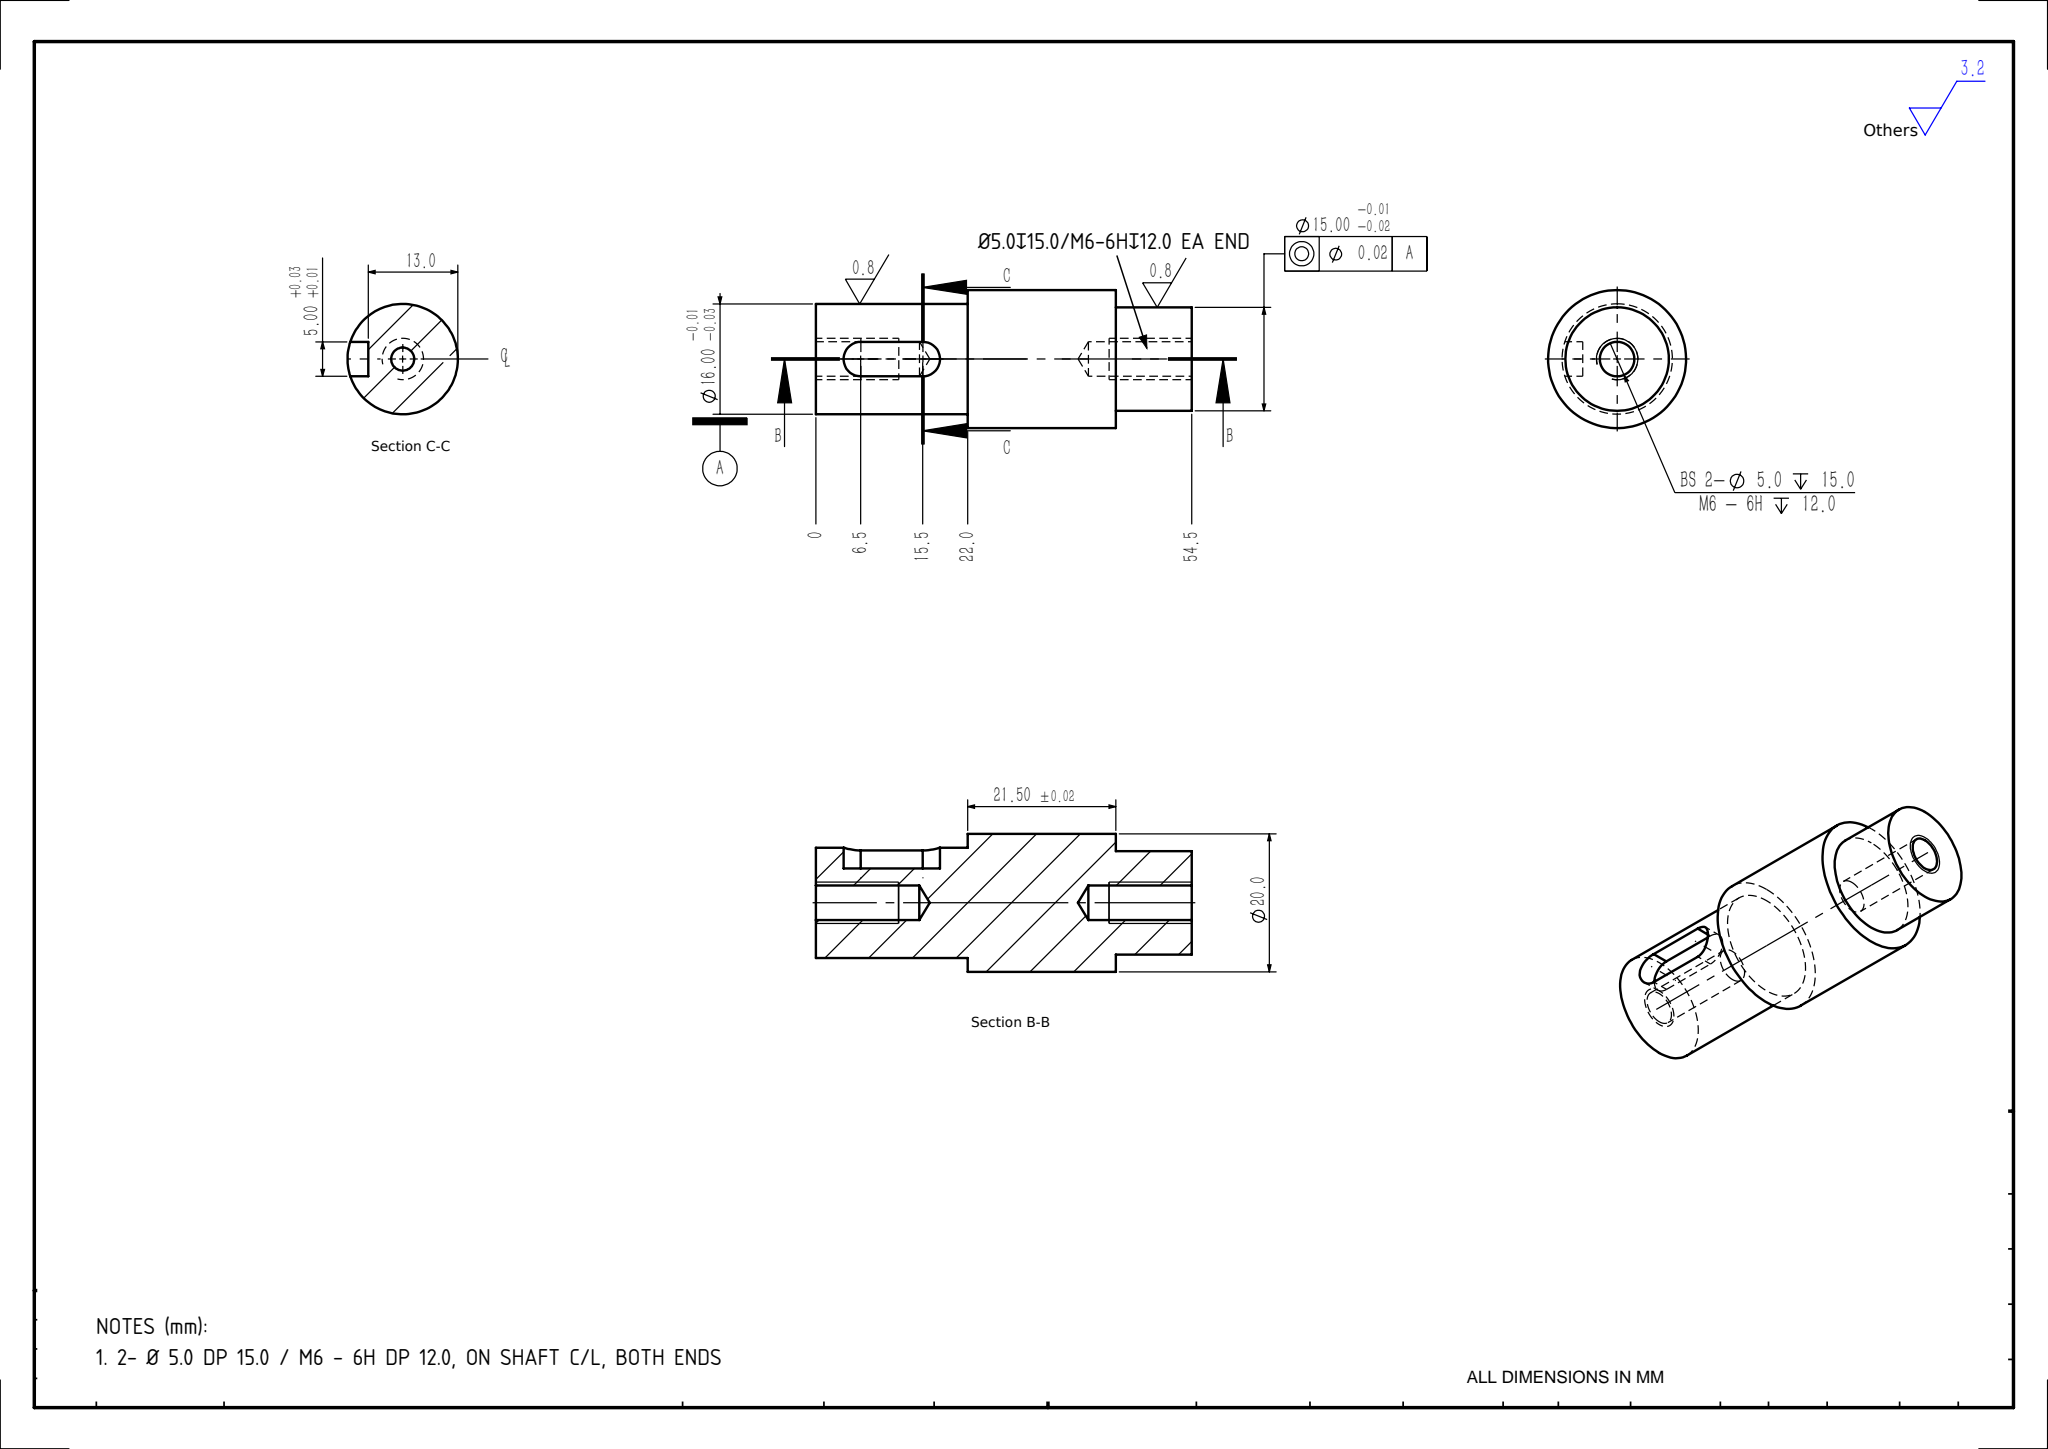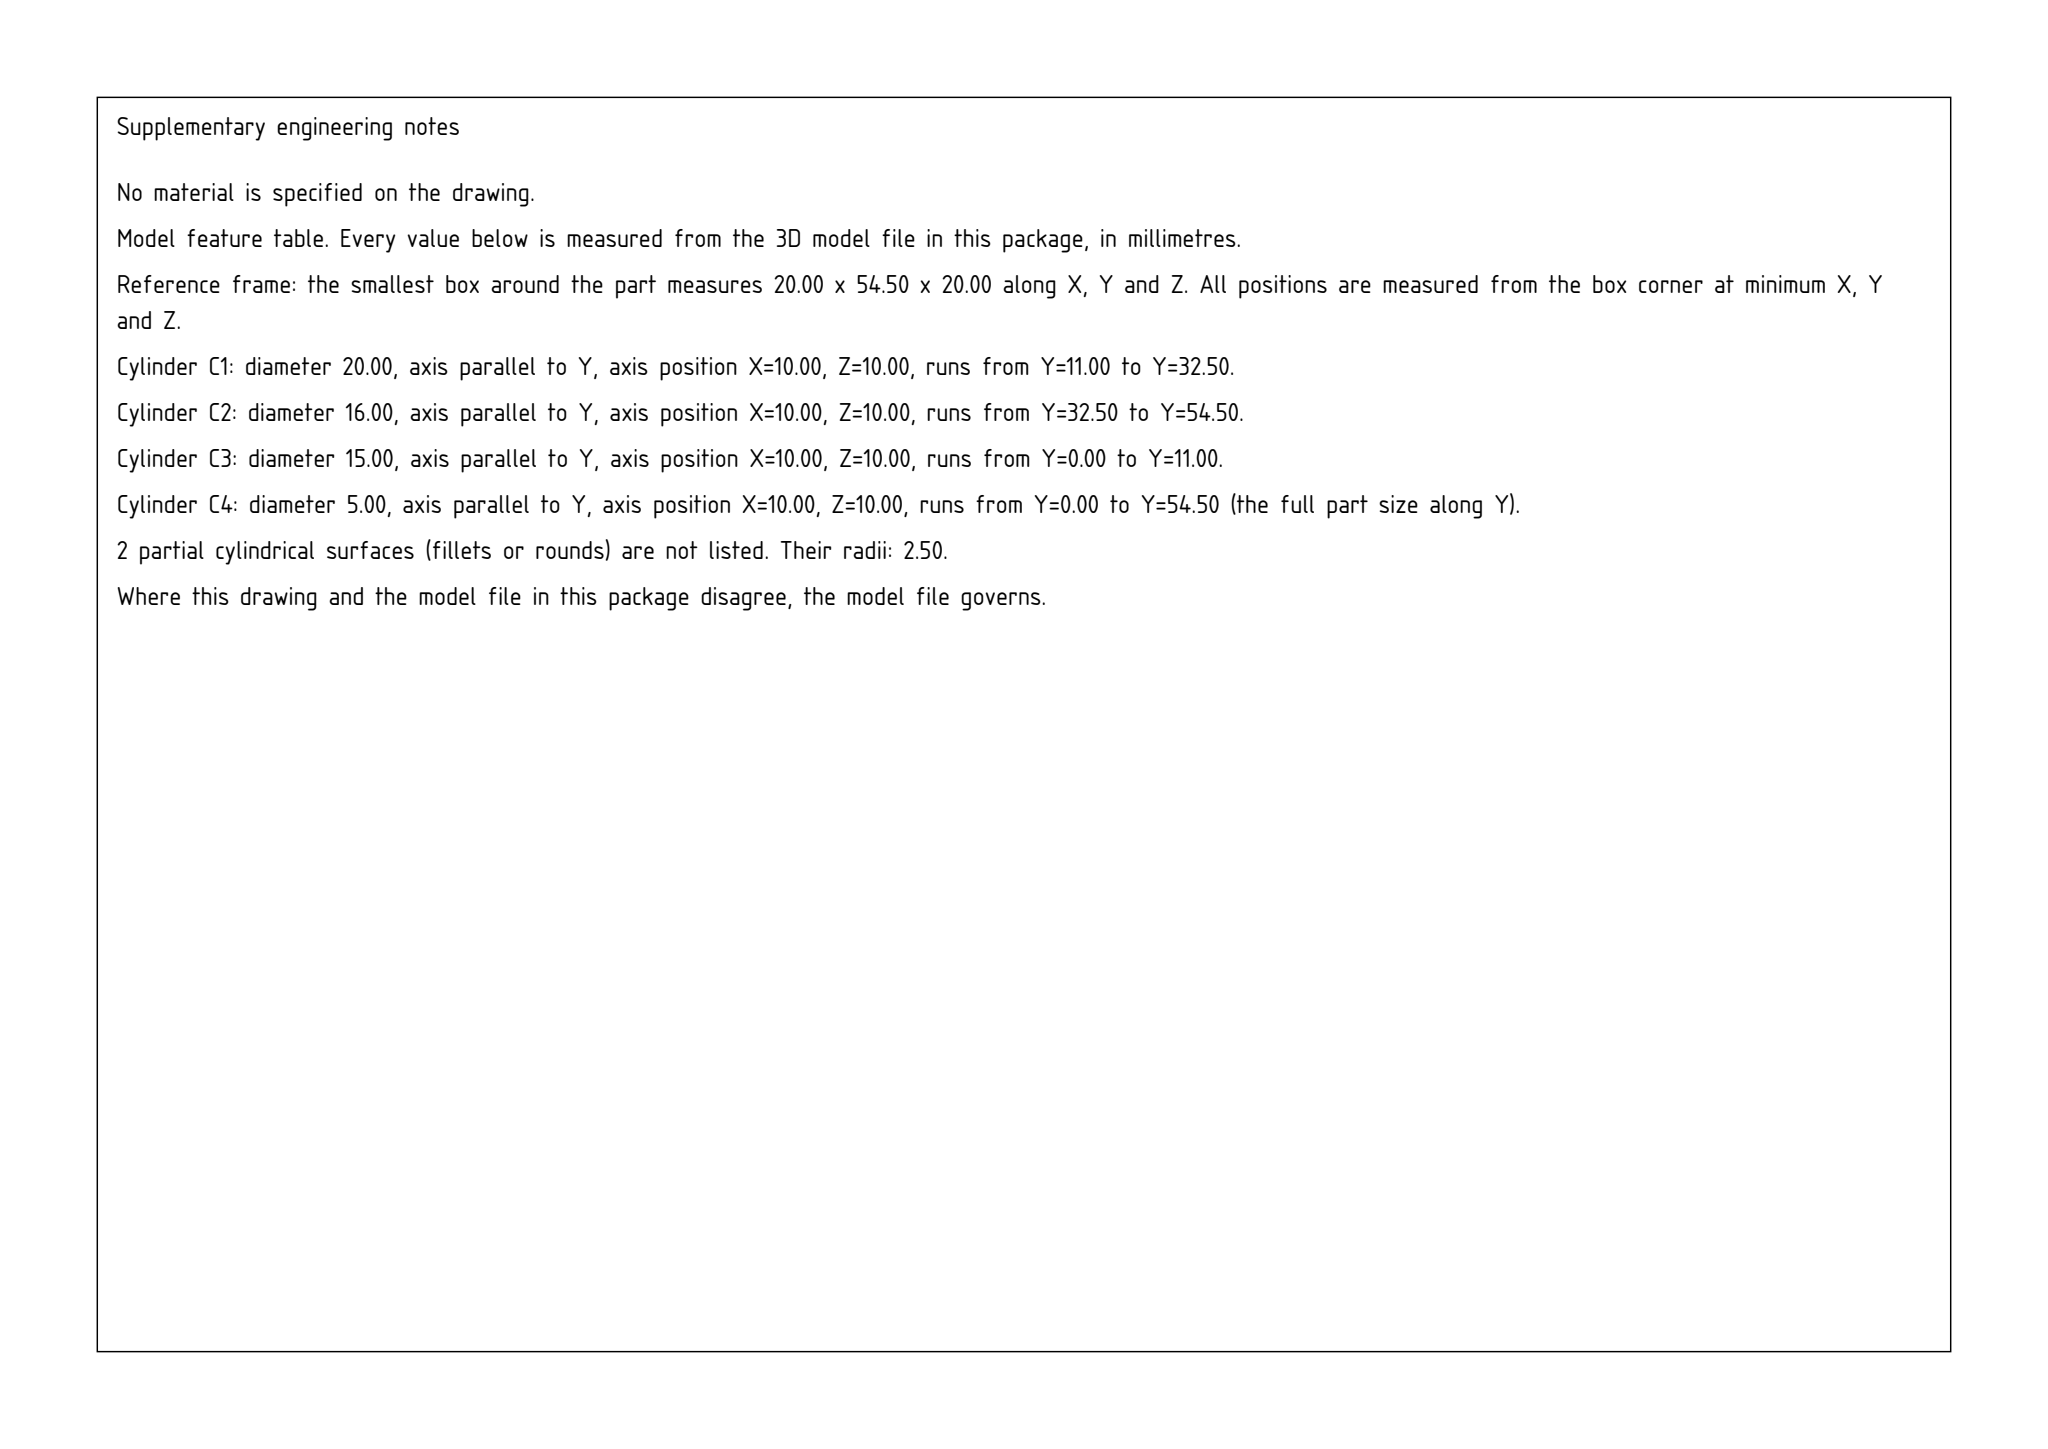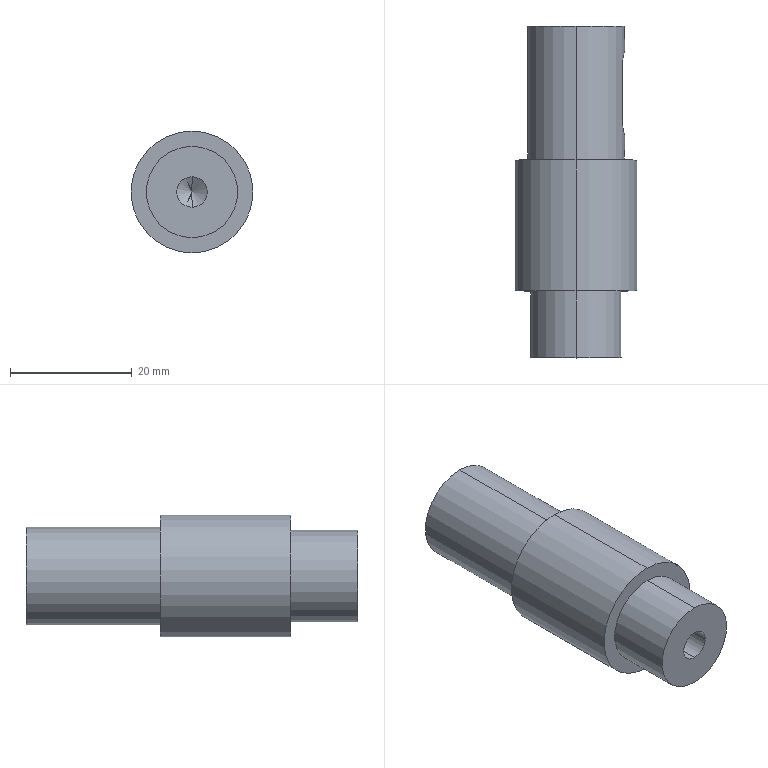Part | SolidWorks | mm | 1 solid | 23 faces | box 20 x 54.5 x 20 mm | volume 12327 mm3 | cylinder 12 | plane 7 | cone 4 | commonest cylinder face diameters 5 x6 15 x2 16 x2 20 x2
Drawing notes:
2- Ø 5.0 DP 15.0 / M6 - 6H DP 12.0, ON SHAFT C/L, BOTH ENDS | from the solid: Two Ø5.0 bores on Y axis at [10,10]: y 0->15 and y 39.5->54.5 (15 deep each), with 118° drill points; threaded M6 depth 12 per callout
2- Ø5.0 DP 15.0 / M6-6H DP 12.0, ONE EA END (DELETE "BS") | from the solid: Two Ø5.0 y-axis bores: y 0.0-15.0 and y 39.5-54.5 (15 deep each), both on axis x=10,z=10; 118° drill points at Ø5.0
build123d program:
from build123d import *

# Parameters (mm, degrees)
SKETCH1_R             = 8
BOSS_EXTRUDE1_DEPTH   = 22
SKETCH2_R             = 10
BOSS_EXTRUDE2_DEPTH   = 32.5
CUT_EXTRUDE1_START    = -11
SKETCH3_R             = 10
SKETCH3_R_2           = 7.5
CUT_EXTRUDE1_DEPTH    = 11
M6_TAPPED_HOLE1_D     = 5
M6_TAPPED_HOLE1_DEPTH = 15
M6_TAPPED_HOLE1_TIP   = 1.502
M6_TAPPED_HOLE2_D     = 5
M6_TAPPED_HOLE2_DEPTH = 15
M6_TAPPED_HOLE2_TIP   = 1.502
CUT_EXTRUDE2_DEPTH    = 3


with BuildPart() as part:
    # Sketch1 → Boss-Extrude1 (new body)
    with BuildSketch(Plane(origin=(0, 0, 0), x_dir=(1, 0, 0), z_dir=(0, 1, 0))):
        with Locations(Location((0, 0, 0), (0, 0, 270))):
            Circle(SKETCH1_R)
    extrude(amount=BOSS_EXTRUDE1_DEPTH)

    # Sketch2 → Boss-Extrude2 (add)
    with BuildSketch(Plane.XZ):
        with Locations(Location((0, 0, 0), (0, 0, 270))):
            Circle(SKETCH2_R)
    extrude(amount=BOSS_EXTRUDE2_DEPTH)

    # Sketch3 → Cut-Extrude1 (cut)
    with BuildSketch(Plane.XZ.offset(32.5).offset(CUT_EXTRUDE1_START)):
        with Locations(Location((0, 0, 0), (0, 0, 270))):
            Circle(SKETCH3_R)
        with Locations(Location((0, 0, 0), (0, 0, 270))):
            Circle(SKETCH3_R_2, mode=Mode.SUBTRACT)
    extrude(amount=CUT_EXTRUDE1_DEPTH, mode=Mode.SUBTRACT)

    # M6 Tapped Hole1
    with Locations(Plane(origin=(0, 22, 0), x_dir=(1, 0, 0), z_dir=(0, 1, 0))):
        with Locations((0, 0)):
            Hole(M6_TAPPED_HOLE1_D / 2, depth=M6_TAPPED_HOLE1_DEPTH)
            with Locations((0, 0, -(M6_TAPPED_HOLE1_DEPTH + M6_TAPPED_HOLE1_TIP / 2))):  # 118° drill point
                Cone(0, M6_TAPPED_HOLE1_D / 2, M6_TAPPED_HOLE1_TIP, mode=Mode.SUBTRACT)

    # M6 Tapped Hole2
    with Locations(Plane(origin=(0, -32.5, 0), x_dir=(-1, 0, 0), z_dir=(0, -1, 0))):
        with Locations((0, 0)):
            Hole(M6_TAPPED_HOLE2_D / 2, depth=M6_TAPPED_HOLE2_DEPTH)
            with Locations((0, 0, -(M6_TAPPED_HOLE2_DEPTH + M6_TAPPED_HOLE2_TIP / 2))):  # 118° drill point
                Cone(0, M6_TAPPED_HOLE2_D / 2, M6_TAPPED_HOLE2_TIP, mode=Mode.SUBTRACT)

    # Sketch11 → Cut-Extrude2 (cut)
    with BuildSketch(Plane(origin=(8, 0, 0), x_dir=(0, 0, -1), z_dir=(1, 0, 0))):
        with BuildLine():
            Line((-2.5, 6.5), (-2.5, 15.5))
            ThreePointArc((-2.5, 15.5), (0, 18), (2.5, 15.5))
            Line((2.5, 15.5), (2.5, 6.5))
            ThreePointArc((2.5, 6.5), (0, 4), (-2.5, 6.5))
        make_face()
    extrude(amount=-CUT_EXTRUDE2_DEPTH, mode=Mode.SUBTRACT)


solid = part.part
STEP:
#1=CARTESIAN_POINT('',(0.,-17.5,2.5));
#2=VERTEX_POINT('',#1);
#3=CARTESIAN_POINT('',(0.,-17.5,-2.5));
#4=VERTEX_POINT('',#3);
#5=CARTESIAN_POINT('',(0.,-17.5,0.));
#6=DIRECTION('',(0.,-1.,0.));
#7=DIRECTION('',(0.,0.,-1.));
#8=AXIS2_PLACEMENT_3D('',#5,#6,#7);
#9=CIRCLE('',#8,2.5);
#10=EDGE_CURVE('',#2,#4,#9,.T.);
#11=ORIENTED_EDGE('',*,*,#10,.F.);
#12=CARTESIAN_POINT('',(0.,-32.5,2.5));
#13=VERTEX_POINT('',#12);
#14=CARTESIAN_POINT('',(0.,-32.5,2.5));
#15=DIRECTION('',(0.,-1.,0.));
#16=VECTOR('',#15,1000.);
#17=LINE('',#14,#16);
#18=EDGE_CURVE('',#2,#13,#17,.T.);
#19=ORIENTED_EDGE('',*,*,#18,.T.);
#20=CARTESIAN_POINT('',(0.,-32.5,-2.5));
#21=VERTEX_POINT('',#20);
#22=CARTESIAN_POINT('',(0.,-32.5,0.));
#23=DIRECTION('',(0.,-1.,0.));
#24=DIRECTION('',(0.,0.,-1.));
#25=AXIS2_PLACEMENT_3D('',#22,#23,#24);
#26=CIRCLE('',#25,2.5);
#27=EDGE_CURVE('',#13,#21,#26,.T.);
#28=ORIENTED_EDGE('',*,*,#27,.T.);
#29=CARTESIAN_POINT('',(0.,-32.5,-2.5));
#30=DIRECTION('',(0.,-1.,0.));
#31=VECTOR('',#30,1000.);
#32=LINE('',#29,#31);
#33=EDGE_CURVE('',#4,#21,#32,.T.);
#34=ORIENTED_EDGE('',*,*,#33,.F.);
#35=EDGE_LOOP('',(#11,#19,#28,#34));
#36=FACE_OUTER_BOUND('',#35,.T.);
#37=CARTESIAN_POINT('',(0.,-32.5,0.));
#38=DIRECTION('',(0.,-1.,0.));
#39=DIRECTION('',(0.,0.,-1.));
#40=AXIS2_PLACEMENT_3D('',#37,#38,#39);
#41=CYLINDRICAL_SURFACE('',#40,2.5);
#42=ADVANCED_FACE('',(#36),#41,.F.);
#43=CARTESIAN_POINT('',(-0.,-15.998,0.));
#44=VERTEX_POINT('',#43);
#45=CARTESIAN_POINT('',(0.,-17.5,-2.5));
#46=DIRECTION('',(0.,-0.515,-0.8572));
#47=VECTOR('',#46,1000.);
#48=LINE('',#45,#47);
#49=EDGE_CURVE('',#44,#4,#48,.T.);
#50=ORIENTED_EDGE('',*,*,#49,.F.);
#51=CARTESIAN_POINT('',(0.,-17.5,2.5));
#52=DIRECTION('',(0.,-0.515,0.8572));
#53=VECTOR('',#52,1000.);
#54=LINE('',#51,#53);
#55=EDGE_CURVE('',#44,#2,#54,.T.);
#56=ORIENTED_EDGE('',*,*,#55,.T.);
#57=ORIENTED_EDGE('',*,*,#10,.T.);
#58=EDGE_LOOP('',(#50,#56,#57));
#59=FACE_OUTER_BOUND('',#58,.T.);
#60=CARTESIAN_POINT('',(0.,-17.5,0.));
#61=DIRECTION('',(0.,-1.,0.));
#62=DIRECTION('',(0.,0.,-1.));
#63=AXIS2_PLACEMENT_3D('',#60,#61,#62);
#64=CONICAL_SURFACE('',#63,2.5,1.03);
#65=ADVANCED_FACE('',(#59),#64,.F.);
#66=CARTESIAN_POINT('',(0.,7.,-2.5));
#67=VERTEX_POINT('',#66);
#68=CARTESIAN_POINT('',(0.,7.,2.5));
#69=VERTEX_POINT('',#68);
#70=CARTESIAN_POINT('',(0.,7.,0.));
#71=DIRECTION('',(0.,1.,0.));
#72=DIRECTION('',(0.,0.,1.));
#73=AXIS2_PLACEMENT_3D('',#70,#71,#72);
#74=CIRCLE('',#73,2.5);
#75=EDGE_CURVE('',#67,#69,#74,.T.);
#76=ORIENTED_EDGE('',*,*,#75,.F.);
#77=CARTESIAN_POINT('',(0.,22.,-2.5));
#78=VERTEX_POINT('',#77);
#79=CARTESIAN_POINT('',(0.,22.,-2.5));
#80=DIRECTION('',(0.,1.,0.));
#81=VECTOR('',#80,1000.);
#82=LINE('',#79,#81);
#83=EDGE_CURVE('',#67,#78,#82,.T.);
#84=ORIENTED_EDGE('',*,*,#83,.T.);
#85=CARTESIAN_POINT('',(0.,22.,2.5));
#86=VERTEX_POINT('',#85);
#87=CARTESIAN_POINT('',(0.,22.,0.));
#88=DIRECTION('',(0.,1.,0.));
#89=DIRECTION('',(0.,0.,1.));
#90=AXIS2_PLACEMENT_3D('',#87,#88,#89);
#91=CIRCLE('',#90,2.5);
#92=EDGE_CURVE('',#78,#86,#91,.T.);
#93=ORIENTED_EDGE('',*,*,#92,.T.);
#94=CARTESIAN_POINT('',(0.,22.,2.5));
#95=DIRECTION('',(0.,1.,0.));
#96=VECTOR('',#95,1000.);
#97=LINE('',#94,#96);
#98=EDGE_CURVE('',#69,#86,#97,.T.);
#99=ORIENTED_EDGE('',*,*,#98,.F.);
#100=EDGE_LOOP('',(#76,#84,#93,#99));
#101=FACE_OUTER_BOUND('',#100,.T.);
#102=CARTESIAN_POINT('',(0.,22.,0.));
#103=DIRECTION('',(0.,1.,0.));
#104=DIRECTION('',(0.,0.,1.));
#105=AXIS2_PLACEMENT_3D('',#102,#103,#104);
#106=CYLINDRICAL_SURFACE('',#105,2.5);
#107=ADVANCED_FACE('',(#101),#106,.F.);
#108=CARTESIAN_POINT('',(-0.,5.498,0.));
#109=VERTEX_POINT('',#108);
#110=CARTESIAN_POINT('',(0.,7.,2.5));
#111=DIRECTION('',(0.,0.515,0.8572));
#112=VECTOR('',#111,1000.);
#113=LINE('',#110,#112);
#114=EDGE_CURVE('',#109,#69,#113,.T.);
#115=ORIENTED_EDGE('',*,*,#114,.F.);
#116=CARTESIAN_POINT('',(0.,7.,-2.5));
#117=DIRECTION('',(0.,0.515,-0.8572));
#118=VECTOR('',#117,1000.);
#119=LINE('',#116,#118);
#120=EDGE_CURVE('',#109,#67,#119,.T.);
#121=ORIENTED_EDGE('',*,*,#120,.T.);
#122=ORIENTED_EDGE('',*,*,#75,.T.);
#123=EDGE_LOOP('',(#115,#121,#122));
#124=FACE_OUTER_BOUND('',#123,.T.);
#125=CARTESIAN_POINT('',(0.,7.,0.));
#126=DIRECTION('',(0.,1.,0.));
#127=DIRECTION('',(0.,0.,1.));
#128=AXIS2_PLACEMENT_3D('',#125,#126,#127);
#129=CONICAL_SURFACE('',#128,2.5,1.03);
#130=ADVANCED_FACE('',(#124),#129,.F.);
#131=CARTESIAN_POINT('',(0.,-21.5,-7.5));
#132=VERTEX_POINT('',#131);
#133=CARTESIAN_POINT('',(0.,-21.5,7.5));
#134=VERTEX_POINT('',#133);
#135=CARTESIAN_POINT('',(0.,-21.5,0.));
#136=DIRECTION('',(0.,-1.,0.));
#137=DIRECTION('',(0.,0.,-1.));
#138=AXIS2_PLACEMENT_3D('',#135,#136,#137);
#139=CIRCLE('',#138,7.5);
#140=EDGE_CURVE('',#132,#134,#139,.T.);
#141=ORIENTED_EDGE('',*,*,#140,.T.);
#142=CARTESIAN_POINT('',(0.,-32.5,7.5));
#143=VERTEX_POINT('',#142);
#144=CARTESIAN_POINT('',(0.,-21.5,7.5));
#145=DIRECTION('',(0.,-1.,0.));
#146=VECTOR('',#145,1000.);
#147=LINE('',#144,#146);
#148=EDGE_CURVE('',#134,#143,#147,.T.);
#149=ORIENTED_EDGE('',*,*,#148,.T.);
#150=CARTESIAN_POINT('',(0.,-32.5,-7.5));
#151=VERTEX_POINT('',#150);
#152=CARTESIAN_POINT('',(0.,-32.5,0.));
#153=DIRECTION('',(0.,-1.,0.));
#154=DIRECTION('',(0.,0.,-1.));
#155=AXIS2_PLACEMENT_3D('',#152,#153,#154);
#156=CIRCLE('',#155,7.5);
#157=EDGE_CURVE('',#151,#143,#156,.T.);
#158=ORIENTED_EDGE('',*,*,#157,.F.);
#159=CARTESIAN_POINT('',(0.,-21.5,-7.5));
#160=DIRECTION('',(0.,-1.,0.));
#161=VECTOR('',#160,1000.);
#162=LINE('',#159,#161);
#163=EDGE_CURVE('',#132,#151,#162,.T.);
#164=ORIENTED_EDGE('',*,*,#163,.F.);
#165=EDGE_LOOP('',(#141,#149,#158,#164));
#166=FACE_OUTER_BOUND('',#165,.T.);
#167=CARTESIAN_POINT('',(0.,-21.5,0.));
#168=DIRECTION('',(0.,-1.,0.));
#169=DIRECTION('',(0.,0.,-1.));
#170=AXIS2_PLACEMENT_3D('',#167,#168,#169);
#171=CYLINDRICAL_SURFACE('',#170,7.5);
#172=ADVANCED_FACE('',(#166),#171,.T.);
#173=CARTESIAN_POINT('',(7.599,6.5,2.5));
#174=VERTEX_POINT('',#173);
#175=CARTESIAN_POINT('',(7.599,15.5,2.5));
#176=VERTEX_POINT('',#175);
#177=CARTESIAN_POINT('',(7.599,22.,2.5));
#178=DIRECTION('',(0.,1.,0.));
#179=VECTOR('',#178,1000.);
#180=LINE('',#177,#179);
#181=EDGE_CURVE('',#174,#176,#180,.T.);
#182=ORIENTED_EDGE('',*,*,#181,.T.);
#183=CARTESIAN_POINT('',(7.599,15.5,-2.5));
#184=VERTEX_POINT('',#183);
#185=CARTESIAN_POINT('',(7.599,15.5,2.5));
#186=CARTESIAN_POINT('',(7.599,15.666,2.5));
#187=CARTESIAN_POINT('',(7.605,15.83,2.484));
#188=CARTESIAN_POINT('',(7.625,16.15,2.419));
#189=CARTESIAN_POINT('',(7.641,16.31,2.371));
#190=CARTESIAN_POINT('',(7.679,16.612,2.245));
#191=CARTESIAN_POINT('',(7.701,16.755,2.168));
#192=CARTESIAN_POINT('',(7.75,17.026,1.987));
#193=CARTESIAN_POINT('',(7.776,17.153,1.882));
#194=CARTESIAN_POINT('',(7.854,17.497,1.539));
#195=CARTESIAN_POINT('',(7.906,17.683,1.262));
#196=CARTESIAN_POINT('',(7.96,17.87,0.8114));
#197=CARTESIAN_POINT('',(7.975,17.919,0.6527));
#198=CARTESIAN_POINT('',(7.995,17.984,0.3296));
#199=CARTESIAN_POINT('',(8.,18.,0.1667));
#200=CARTESIAN_POINT('',(8.,18.,-0.1617));
#201=CARTESIAN_POINT('',(7.995,17.984,-0.3285));
#202=CARTESIAN_POINT('',(7.975,17.92,-0.6499));
#203=CARTESIAN_POINT('',(7.961,17.872,-0.8063));
#204=CARTESIAN_POINT('',(7.924,17.746,-1.11));
#205=CARTESIAN_POINT('',(7.902,17.668,-1.255));
#206=CARTESIAN_POINT('',(7.855,17.488,-1.525));
#207=CARTESIAN_POINT('',(7.828,17.383,-1.652));
#208=CARTESIAN_POINT('',(7.776,17.153,-1.883));
#209=CARTESIAN_POINT('',(7.75,17.028,-1.985));
#210=CARTESIAN_POINT('',(7.702,16.758,-2.166));
#211=CARTESIAN_POINT('',(7.679,16.612,-2.245));
#212=CARTESIAN_POINT('',(7.641,16.311,-2.37));
#213=CARTESIAN_POINT('',(7.626,16.155,-2.418));
#214=CARTESIAN_POINT('',(7.605,15.832,-2.483));
#215=CARTESIAN_POINT('',(7.599,15.666,-2.5));
#216=CARTESIAN_POINT('',(7.599,15.5,-2.5));
#217=B_SPLINE_CURVE_WITH_KNOTS('',3,(#185,#186,#187,#188,#189,#190,#191,#192,#193,#194,#195,#196,#197,#198,#199,#200,#201,#202,#203,#204,#205,#206,#207,#208,#209,#210,#211,#212,#213,#214,#215,#216),.UNSPECIFIED.,.F.,.F.,(4,2,2,2,2,2,2,2,2,2,2,2,2,2,2,4),(0.,0.0004914,0.0009828,0.001474,0.001966,0.002949,0.00344,0.003931,0.004423,0.004914,0.005406,0.005897,0.006388,0.00688,0.007371,0.007863),.UNSPECIFIED.);
#218=EDGE_CURVE('',#176,#184,#217,.T.);
#219=ORIENTED_EDGE('',*,*,#218,.T.);
#220=CARTESIAN_POINT('',(7.599,6.5,-2.5));
#221=VERTEX_POINT('',#220);
#222=CARTESIAN_POINT('',(7.599,22.,-2.5));
#223=DIRECTION('',(0.,-1.,0.));
#224=VECTOR('',#223,1000.);
#225=LINE('',#222,#224);
#226=EDGE_CURVE('',#184,#221,#225,.T.);
#227=ORIENTED_EDGE('',*,*,#226,.T.);
#228=CARTESIAN_POINT('',(7.599,6.5,-2.5));
#229=CARTESIAN_POINT('',(7.599,6.334,-2.5));
#230=CARTESIAN_POINT('',(7.605,6.17,-2.484));
#231=CARTESIAN_POINT('',(7.625,5.85,-2.419));
#232=CARTESIAN_POINT('',(7.641,5.69,-2.371));
#233=CARTESIAN_POINT('',(7.679,5.388,-2.245));
#234=CARTESIAN_POINT('',(7.701,5.245,-2.168));
#235=CARTESIAN_POINT('',(7.75,4.974,-1.987));
#236=CARTESIAN_POINT('',(7.776,4.847,-1.882));
#237=CARTESIAN_POINT('',(7.854,4.503,-1.539));
#238=CARTESIAN_POINT('',(7.906,4.317,-1.262));
#239=CARTESIAN_POINT('',(7.96,4.13,-0.8114));
#240=CARTESIAN_POINT('',(7.975,4.081,-0.6527));
#241=CARTESIAN_POINT('',(7.995,4.016,-0.3296));
#242=CARTESIAN_POINT('',(8.,4.,-0.1667));
#243=CARTESIAN_POINT('',(8.,4.,0.1617));
#244=CARTESIAN_POINT('',(7.995,4.016,0.3285));
#245=CARTESIAN_POINT('',(7.975,4.08,0.6499));
#246=CARTESIAN_POINT('',(7.961,4.128,0.8063));
#247=CARTESIAN_POINT('',(7.924,4.254,1.11));
#248=CARTESIAN_POINT('',(7.902,4.332,1.255));
#249=CARTESIAN_POINT('',(7.855,4.512,1.525));
#250=CARTESIAN_POINT('',(7.828,4.617,1.652));
#251=CARTESIAN_POINT('',(7.776,4.847,1.883));
#252=CARTESIAN_POINT('',(7.75,4.972,1.985));
#253=CARTESIAN_POINT('',(7.702,5.242,2.166));
#254=CARTESIAN_POINT('',(7.679,5.388,2.245));
#255=CARTESIAN_POINT('',(7.641,5.689,2.37));
#256=CARTESIAN_POINT('',(7.626,5.845,2.418));
#257=CARTESIAN_POINT('',(7.605,6.168,2.483));
#258=CARTESIAN_POINT('',(7.599,6.334,2.5));
#259=CARTESIAN_POINT('',(7.599,6.5,2.5));
#260=B_SPLINE_CURVE_WITH_KNOTS('',3,(#228,#229,#230,#231,#232,#233,#234,#235,#236,#237,#238,#239,#240,#241,#242,#243,#244,#245,#246,#247,#248,#249,#250,#251,#252,#253,#254,#255,#256,#257,#258,#259),.UNSPECIFIED.,.F.,.F.,(4,2,2,2,2,2,2,2,2,2,2,2,2,2,2,4),(0.,0.0004914,0.0009828,0.001474,0.001966,0.002949,0.00344,0.003931,0.004423,0.004914,0.005406,0.005897,0.006388,0.00688,0.007371,0.007863),.UNSPECIFIED.);
#261=EDGE_CURVE('',#221,#174,#260,.T.);
#262=ORIENTED_EDGE('',*,*,#261,.T.);
#263=EDGE_LOOP('',(#182,#219,#227,#262));
#264=FACE_BOUND('',#263,.T.);
#265=CARTESIAN_POINT('',(0.,22.,8.));
#266=VERTEX_POINT('',#265);
#267=CARTESIAN_POINT('',(0.,22.,-8.));
#268=VERTEX_POINT('',#267);
#269=CARTESIAN_POINT('',(0.,22.,0.));
#270=DIRECTION('',(0.,1.,0.));
#271=DIRECTION('',(0.,0.,1.));
#272=AXIS2_PLACEMENT_3D('',#269,#270,#271);
#273=CIRCLE('',#272,8.);
#274=EDGE_CURVE('',#266,#268,#273,.T.);
#275=ORIENTED_EDGE('',*,*,#274,.F.);
#276=CARTESIAN_POINT('',(0.,0.,8.));
#277=VERTEX_POINT('',#276);
#278=CARTESIAN_POINT('',(0.,22.,8.));
#279=DIRECTION('',(0.,-1.,0.));
#280=VECTOR('',#279,1000.);
#281=LINE('',#278,#280);
#282=EDGE_CURVE('',#266,#277,#281,.T.);
#283=ORIENTED_EDGE('',*,*,#282,.T.);
#284=CARTESIAN_POINT('',(0.,0.,-8.));
#285=VERTEX_POINT('',#284);
#286=CARTESIAN_POINT('',(0.,0.,0.));
#287=DIRECTION('',(0.,-1.,0.));
#288=DIRECTION('',(0.,0.,-1.));
#289=AXIS2_PLACEMENT_3D('',#286,#287,#288);
#290=CIRCLE('',#289,8.);
#291=EDGE_CURVE('',#285,#277,#290,.T.);
#292=ORIENTED_EDGE('',*,*,#291,.F.);
#293=CARTESIAN_POINT('',(0.,22.,-8.));
#294=DIRECTION('',(0.,-1.,0.));
#295=VECTOR('',#294,1000.);
#296=LINE('',#293,#295);
#297=EDGE_CURVE('',#268,#285,#296,.T.);
#298=ORIENTED_EDGE('',*,*,#297,.F.);
#299=EDGE_LOOP('',(#275,#283,#292,#298));
#300=FACE_OUTER_BOUND('',#299,.T.);
#301=CARTESIAN_POINT('',(0.,22.,0.));
#302=DIRECTION('',(0.,-1.,0.));
#303=DIRECTION('',(0.,0.,-1.));
#304=AXIS2_PLACEMENT_3D('',#301,#302,#303);
#305=CYLINDRICAL_SURFACE('',#304,8.);
#306=ADVANCED_FACE('',(#264,#300),#305,.T.);
#307=CARTESIAN_POINT('',(0.,-21.5,-10.));
#308=VERTEX_POINT('',#307);
#309=CARTESIAN_POINT('',(0.,-21.5,10.));
#310=VERTEX_POINT('',#309);
#311=CARTESIAN_POINT('',(0.,-21.5,0.));
#312=DIRECTION('',(0.,-1.,0.));
#313=DIRECTION('',(0.,0.,-1.));
#314=AXIS2_PLACEMENT_3D('',#311,#312,#313);
#315=CIRCLE('',#314,10.);
#316=EDGE_CURVE('',#308,#310,#315,.T.);
#317=ORIENTED_EDGE('',*,*,#316,.F.);
#318=CARTESIAN_POINT('',(0.,0.,-10.));
#319=VERTEX_POINT('',#318);
#320=CARTESIAN_POINT('',(0.,-32.5,-10.));
#321=DIRECTION('',(0.,1.,0.));
#322=VECTOR('',#321,1000.);
#323=LINE('',#320,#322);
#324=EDGE_CURVE('',#308,#319,#323,.T.);
#325=ORIENTED_EDGE('',*,*,#324,.T.);
#326=CARTESIAN_POINT('',(0.,0.,10.));
#327=VERTEX_POINT('',#326);
#328=CARTESIAN_POINT('',(0.,0.,0.));
#329=DIRECTION('',(0.,-1.,0.));
#330=DIRECTION('',(0.,0.,-1.));
#331=AXIS2_PLACEMENT_3D('',#328,#329,#330);
#332=CIRCLE('',#331,10.);
#333=EDGE_CURVE('',#319,#327,#332,.T.);
#334=ORIENTED_EDGE('',*,*,#333,.T.);
#335=CARTESIAN_POINT('',(0.,-32.5,10.));
#336=DIRECTION('',(0.,1.,0.));
#337=VECTOR('',#336,1000.);
#338=LINE('',#335,#337);
#339=EDGE_CURVE('',#310,#327,#338,.T.);
#340=ORIENTED_EDGE('',*,*,#339,.F.);
#341=EDGE_LOOP('',(#317,#325,#334,#340));
#342=FACE_OUTER_BOUND('',#341,.T.);
#343=CARTESIAN_POINT('',(0.,-32.5,0.));
#344=DIRECTION('',(0.,1.,0.));
#345=DIRECTION('',(0.,0.,1.));
#346=AXIS2_PLACEMENT_3D('',#343,#344,#345);
#347=CYLINDRICAL_SURFACE('',#346,10.);
#348=ADVANCED_FACE('',(#342),#347,.T.);
#349=ORIENTED_EDGE('',*,*,#324,.F.);
#350=CARTESIAN_POINT('',(0.,-21.5,0.));
#351=DIRECTION('',(0.,-1.,0.));
#352=DIRECTION('',(0.,0.,-1.));
#353=AXIS2_PLACEMENT_3D('',#350,#351,#352);
#354=CIRCLE('',#353,10.);
#355=EDGE_CURVE('',#310,#308,#354,.T.);
#356=ORIENTED_EDGE('',*,*,#355,.F.);
#357=ORIENTED_EDGE('',*,*,#339,.T.);
#358=CARTESIAN_POINT('',(0.,0.,0.));
#359=DIRECTION('',(0.,-1.,0.));
#360=DIRECTION('',(0.,0.,-1.));
#361=AXIS2_PLACEMENT_3D('',#358,#359,#360);
#362=CIRCLE('',#361,10.);
#363=EDGE_CURVE('',#327,#319,#362,.T.);
#364=ORIENTED_EDGE('',*,*,#363,.T.);
#365=EDGE_LOOP('',(#349,#356,#357,#364));
#366=FACE_OUTER_BOUND('',#365,.T.);
#367=CARTESIAN_POINT('',(0.,-32.5,0.));
#368=DIRECTION('',(0.,1.,0.));
#369=DIRECTION('',(0.,0.,1.));
#370=AXIS2_PLACEMENT_3D('',#367,#368,#369);
#371=CYLINDRICAL_SURFACE('',#370,10.);
#372=ADVANCED_FACE('',(#366),#371,.T.);
#373=ORIENTED_EDGE('',*,*,#282,.F.);
#374=CARTESIAN_POINT('',(0.,22.,0.));
#375=DIRECTION('',(0.,1.,0.));
#376=DIRECTION('',(0.,0.,1.));
#377=AXIS2_PLACEMENT_3D('',#374,#375,#376);
#378=CIRCLE('',#377,8.);
#379=EDGE_CURVE('',#268,#266,#378,.T.);
#380=ORIENTED_EDGE('',*,*,#379,.F.);
#381=ORIENTED_EDGE('',*,*,#297,.T.);
#382=CARTESIAN_POINT('',(0.,0.,0.));
#383=DIRECTION('',(0.,-1.,0.));
#384=DIRECTION('',(0.,0.,-1.));
#385=AXIS2_PLACEMENT_3D('',#382,#383,#384);
#386=CIRCLE('',#385,8.);
#387=EDGE_CURVE('',#277,#285,#386,.T.);
#388=ORIENTED_EDGE('',*,*,#387,.F.);
#389=EDGE_LOOP('',(#373,#380,#381,#388));
#390=FACE_OUTER_BOUND('',#389,.T.);
#391=CARTESIAN_POINT('',(0.,22.,0.));
#392=DIRECTION('',(0.,-1.,0.));
#393=DIRECTION('',(0.,0.,-1.));
#394=AXIS2_PLACEMENT_3D('',#391,#392,#393);
#395=CYLINDRICAL_SURFACE('',#394,8.);
#396=ADVANCED_FACE('',(#390),#395,.T.);
#397=CARTESIAN_POINT('',(0.,22.,0.));
#398=DIRECTION('',(0.,1.,0.));
#399=DIRECTION('',(0.,0.,1.));
#400=AXIS2_PLACEMENT_3D('',#397,#398,#399);
#401=CIRCLE('',#400,2.5);
#402=EDGE_CURVE('',#86,#78,#401,.T.);
#403=ORIENTED_EDGE('',*,*,#402,.F.);
#404=ORIENTED_EDGE('',*,*,#92,.F.);
#405=EDGE_LOOP('',(#403,#404));
#406=FACE_BOUND('',#405,.T.);
#407=ORIENTED_EDGE('',*,*,#379,.T.);
#408=ORIENTED_EDGE('',*,*,#274,.T.);
#409=EDGE_LOOP('',(#407,#408));
#410=FACE_OUTER_BOUND('',#409,.T.);
#411=CARTESIAN_POINT('',(0.,22.,0.));
#412=DIRECTION('',(0.,1.,0.));
#413=DIRECTION('',(0.,0.,1.));
#414=AXIS2_PLACEMENT_3D('',#411,#412,#413);
#415=PLANE('',#414);
#416=ADVANCED_FACE('',(#406,#410),#415,.T.);
#417=ORIENTED_EDGE('',*,*,#291,.T.);
#418=ORIENTED_EDGE('',*,*,#387,.T.);
#419=EDGE_LOOP('',(#417,#418));
#420=FACE_BOUND('',#419,.T.);
#421=ORIENTED_EDGE('',*,*,#363,.F.);
#422=ORIENTED_EDGE('',*,*,#333,.F.);
#423=EDGE_LOOP('',(#421,#422));
#424=FACE_OUTER_BOUND('',#423,.T.);
#425=CARTESIAN_POINT('',(0.,0.,0.));
#426=DIRECTION('',(0.,-1.,0.));
#427=DIRECTION('',(0.,0.,-1.));
#428=AXIS2_PLACEMENT_3D('',#425,#426,#427);
#429=PLANE('',#428);
#430=ADVANCED_FACE('',(#420,#424),#429,.F.);
#431=ORIENTED_EDGE('',*,*,#140,.F.);
#432=CARTESIAN_POINT('',(0.,-21.5,0.));
#433=DIRECTION('',(0.,-1.,0.));
#434=DIRECTION('',(0.,0.,-1.));
#435=AXIS2_PLACEMENT_3D('',#432,#433,#434);
#436=CIRCLE('',#435,7.5);
#437=EDGE_CURVE('',#134,#132,#436,.T.);
#438=ORIENTED_EDGE('',*,*,#437,.F.);
#439=EDGE_LOOP('',(#431,#438));
#440=FACE_BOUND('',#439,.T.);
#441=ORIENTED_EDGE('',*,*,#355,.T.);
#442=ORIENTED_EDGE('',*,*,#316,.T.);
#443=EDGE_LOOP('',(#441,#442));
#444=FACE_OUTER_BOUND('',#443,.T.);
#445=CARTESIAN_POINT('',(0.,-21.5,0.));
#446=DIRECTION('',(0.,-1.,0.));
#447=DIRECTION('',(0.,0.,-1.));
#448=AXIS2_PLACEMENT_3D('',#445,#446,#447);
#449=PLANE('',#448);
#450=ADVANCED_FACE('',(#440,#444),#449,.T.);
#451=ORIENTED_EDGE('',*,*,#148,.F.);
#452=ORIENTED_EDGE('',*,*,#437,.T.);
#453=ORIENTED_EDGE('',*,*,#163,.T.);
#454=CARTESIAN_POINT('',(0.,-32.5,0.));
#455=DIRECTION('',(0.,-1.,0.));
#456=DIRECTION('',(0.,0.,-1.));
#457=AXIS2_PLACEMENT_3D('',#454,#455,#456);
#458=CIRCLE('',#457,7.5);
#459=EDGE_CURVE('',#143,#151,#458,.T.);
#460=ORIENTED_EDGE('',*,*,#459,.F.);
#461=EDGE_LOOP('',(#451,#452,#453,#460));
#462=FACE_OUTER_BOUND('',#461,.T.);
#463=CARTESIAN_POINT('',(0.,-21.5,0.));
#464=DIRECTION('',(0.,-1.,0.));
#465=DIRECTION('',(0.,0.,-1.));
#466=AXIS2_PLACEMENT_3D('',#463,#464,#465);
#467=CYLINDRICAL_SURFACE('',#466,7.5);
#468=ADVANCED_FACE('',(#462),#467,.T.);
#469=CARTESIAN_POINT('',(0.,-32.5,0.));
#470=DIRECTION('',(0.,-1.,0.));
#471=DIRECTION('',(0.,0.,-1.));
#472=AXIS2_PLACEMENT_3D('',#469,#470,#471);
#473=CIRCLE('',#472,2.5);
#474=EDGE_CURVE('',#21,#13,#473,.T.);
#475=ORIENTED_EDGE('',*,*,#474,.F.);
#476=ORIENTED_EDGE('',*,*,#27,.F.);
#477=EDGE_LOOP('',(#475,#476));
#478=FACE_BOUND('',#477,.T.);
#479=ORIENTED_EDGE('',*,*,#157,.T.);
#480=ORIENTED_EDGE('',*,*,#459,.T.);
#481=EDGE_LOOP('',(#479,#480));
#482=FACE_OUTER_BOUND('',#481,.T.);
#483=CARTESIAN_POINT('',(0.,-32.5,0.));
#484=DIRECTION('',(0.,-1.,0.));
#485=DIRECTION('',(0.,0.,-1.));
#486=AXIS2_PLACEMENT_3D('',#483,#484,#485);
#487=PLANE('',#486);
#488=ADVANCED_FACE('',(#478,#482),#487,.T.);
#489=ORIENTED_EDGE('',*,*,#120,.F.);
#490=ORIENTED_EDGE('',*,*,#114,.T.);
#491=CARTESIAN_POINT('',(0.,7.,0.));
#492=DIRECTION('',(0.,1.,0.));
#493=DIRECTION('',(0.,0.,1.));
#494=AXIS2_PLACEMENT_3D('',#491,#492,#493);
#495=CIRCLE('',#494,2.5);
#496=EDGE_CURVE('',#69,#67,#495,.T.);
#497=ORIENTED_EDGE('',*,*,#496,.T.);
#498=EDGE_LOOP('',(#489,#490,#497));
#499=FACE_OUTER_BOUND('',#498,.T.);
#500=CARTESIAN_POINT('',(0.,7.,0.));
#501=DIRECTION('',(0.,1.,0.));
#502=DIRECTION('',(0.,0.,1.));
#503=AXIS2_PLACEMENT_3D('',#500,#501,#502);
#504=CONICAL_SURFACE('',#503,2.5,1.03);
#505=ADVANCED_FACE('',(#499),#504,.F.);
#506=ORIENTED_EDGE('',*,*,#83,.F.);
#507=ORIENTED_EDGE('',*,*,#496,.F.);
#508=ORIENTED_EDGE('',*,*,#98,.T.);
#509=ORIENTED_EDGE('',*,*,#402,.T.);
#510=EDGE_LOOP('',(#506,#507,#508,#509));
#511=FACE_OUTER_BOUND('',#510,.T.);
#512=CARTESIAN_POINT('',(0.,22.,0.));
#513=DIRECTION('',(0.,1.,0.));
#514=DIRECTION('',(0.,0.,1.));
#515=AXIS2_PLACEMENT_3D('',#512,#513,#514);
#516=CYLINDRICAL_SURFACE('',#515,2.5);
#517=ADVANCED_FACE('',(#511),#516,.F.);
#518=ORIENTED_EDGE('',*,*,#55,.F.);
#519=ORIENTED_EDGE('',*,*,#49,.T.);
#520=CARTESIAN_POINT('',(0.,-17.5,0.));
#521=DIRECTION('',(0.,-1.,0.));
#522=DIRECTION('',(0.,0.,-1.));
#523=AXIS2_PLACEMENT_3D('',#520,#521,#522);
#524=CIRCLE('',#523,2.5);
#525=EDGE_CURVE('',#4,#2,#524,.T.);
#526=ORIENTED_EDGE('',*,*,#525,.T.);
#527=EDGE_LOOP('',(#518,#519,#526));
#528=FACE_OUTER_BOUND('',#527,.T.);
#529=CARTESIAN_POINT('',(0.,-17.5,0.));
#530=DIRECTION('',(0.,-1.,0.));
#531=DIRECTION('',(0.,0.,-1.));
#532=AXIS2_PLACEMENT_3D('',#529,#530,#531);
#533=CONICAL_SURFACE('',#532,2.5,1.03);
#534=ADVANCED_FACE('',(#528),#533,.F.);
#535=ORIENTED_EDGE('',*,*,#18,.F.);
#536=ORIENTED_EDGE('',*,*,#525,.F.);
#537=ORIENTED_EDGE('',*,*,#33,.T.);
#538=ORIENTED_EDGE('',*,*,#474,.T.);
#539=EDGE_LOOP('',(#535,#536,#537,#538));
#540=FACE_OUTER_BOUND('',#539,.T.);
#541=CARTESIAN_POINT('',(0.,-32.5,0.));
#542=DIRECTION('',(0.,-1.,0.));
#543=DIRECTION('',(0.,0.,-1.));
#544=AXIS2_PLACEMENT_3D('',#541,#542,#543);
#545=CYLINDRICAL_SURFACE('',#544,2.5);
#546=ADVANCED_FACE('',(#540),#545,.F.);
#547=CARTESIAN_POINT('',(5.,6.5,-2.5));
#548=VERTEX_POINT('',#547);
#549=CARTESIAN_POINT('',(5.,6.5,-2.5));
#550=DIRECTION('',(1.,0.,0.));
#551=VECTOR('',#550,1000.);
#552=LINE('',#549,#551);
#553=EDGE_CURVE('',#548,#221,#552,.T.);
#554=ORIENTED_EDGE('',*,*,#553,.F.);
#555=CARTESIAN_POINT('',(5.,6.5,2.5));
#556=VERTEX_POINT('',#555);
#557=CARTESIAN_POINT('',(5.,6.5,0.));
#558=DIRECTION('',(1.,0.,0.));
#559=DIRECTION('',(0.,0.,-1.));
#560=AXIS2_PLACEMENT_3D('',#557,#558,#559);
#561=CIRCLE('',#560,2.5);
#562=EDGE_CURVE('',#556,#548,#561,.T.);
#563=ORIENTED_EDGE('',*,*,#562,.F.);
#564=CARTESIAN_POINT('',(5.,6.5,2.5));
#565=DIRECTION('',(1.,0.,0.));
#566=VECTOR('',#565,1000.);
#567=LINE('',#564,#566);
#568=EDGE_CURVE('',#556,#174,#567,.T.);
#569=ORIENTED_EDGE('',*,*,#568,.T.);
#570=ORIENTED_EDGE('',*,*,#261,.F.);
#571=EDGE_LOOP('',(#554,#563,#569,#570));
#572=FACE_OUTER_BOUND('',#571,.T.);
#573=CARTESIAN_POINT('',(5.,6.5,0.));
#574=DIRECTION('',(1.,0.,0.));
#575=DIRECTION('',(0.,0.,-1.));
#576=AXIS2_PLACEMENT_3D('',#573,#574,#575);
#577=CYLINDRICAL_SURFACE('',#576,2.5);
#578=ADVANCED_FACE('',(#572),#577,.F.);
#579=ORIENTED_EDGE('',*,*,#568,.F.);
#580=CARTESIAN_POINT('',(5.,15.5,2.5));
#581=VERTEX_POINT('',#580);
#582=CARTESIAN_POINT('',(5.,6.5,2.5));
#583=DIRECTION('',(0.,-1.,0.));
#584=VECTOR('',#583,1000.);
#585=LINE('',#582,#584);
#586=EDGE_CURVE('',#581,#556,#585,.T.);
#587=ORIENTED_EDGE('',*,*,#586,.F.);
#588=CARTESIAN_POINT('',(5.,15.5,2.5));
#589=DIRECTION('',(1.,0.,0.));
#590=VECTOR('',#589,1000.);
#591=LINE('',#588,#590);
#592=EDGE_CURVE('',#581,#176,#591,.T.);
#593=ORIENTED_EDGE('',*,*,#592,.T.);
#594=ORIENTED_EDGE('',*,*,#181,.F.);
#595=EDGE_LOOP('',(#579,#587,#593,#594));
#596=FACE_OUTER_BOUND('',#595,.T.);
#597=CARTESIAN_POINT('',(5.,6.5,2.5));
#598=DIRECTION('',(0.,0.,1.));
#599=DIRECTION('',(1.,0.,0.));
#600=AXIS2_PLACEMENT_3D('',#597,#598,#599);
#601=PLANE('',#600);
#602=ADVANCED_FACE('',(#596),#601,.F.);
#603=ORIENTED_EDGE('',*,*,#592,.F.);
#604=CARTESIAN_POINT('',(5.,15.5,-2.5));
#605=VERTEX_POINT('',#604);
#606=CARTESIAN_POINT('',(5.,15.5,0.));
#607=DIRECTION('',(1.,0.,0.));
#608=DIRECTION('',(0.,0.,-1.));
#609=AXIS2_PLACEMENT_3D('',#606,#607,#608);
#610=CIRCLE('',#609,2.5);
#611=EDGE_CURVE('',#605,#581,#610,.T.);
#612=ORIENTED_EDGE('',*,*,#611,.F.);
#613=CARTESIAN_POINT('',(5.,15.5,-2.5));
#614=DIRECTION('',(1.,0.,0.));
#615=VECTOR('',#614,1000.);
#616=LINE('',#613,#615);
#617=EDGE_CURVE('',#605,#184,#616,.T.);
#618=ORIENTED_EDGE('',*,*,#617,.T.);
#619=ORIENTED_EDGE('',*,*,#218,.F.);
#620=EDGE_LOOP('',(#603,#612,#618,#619));
#621=FACE_OUTER_BOUND('',#620,.T.);
#622=CARTESIAN_POINT('',(5.,15.5,0.));
#623=DIRECTION('',(1.,0.,0.));
#624=DIRECTION('',(0.,0.,-1.));
#625=AXIS2_PLACEMENT_3D('',#622,#623,#624);
#626=CYLINDRICAL_SURFACE('',#625,2.5);
#627=ADVANCED_FACE('',(#621),#626,.F.);
#628=ORIENTED_EDGE('',*,*,#617,.F.);
#629=CARTESIAN_POINT('',(5.,6.5,-2.5));
#630=DIRECTION('',(0.,1.,0.));
#631=VECTOR('',#630,1000.);
#632=LINE('',#629,#631);
#633=EDGE_CURVE('',#548,#605,#632,.T.);
#634=ORIENTED_EDGE('',*,*,#633,.F.);
#635=ORIENTED_EDGE('',*,*,#553,.T.);
#636=ORIENTED_EDGE('',*,*,#226,.F.);
#637=EDGE_LOOP('',(#628,#634,#635,#636));
#638=FACE_OUTER_BOUND('',#637,.T.);
#639=CARTESIAN_POINT('',(5.,6.5,-2.5));
#640=DIRECTION('',(0.,0.,-1.));
#641=DIRECTION('',(-1.,0.,0.));
#642=AXIS2_PLACEMENT_3D('',#639,#640,#641);
#643=PLANE('',#642);
#644=ADVANCED_FACE('',(#638),#643,.F.);
#645=ORIENTED_EDGE('',*,*,#562,.T.);
#646=ORIENTED_EDGE('',*,*,#633,.T.);
#647=ORIENTED_EDGE('',*,*,#611,.T.);
#648=ORIENTED_EDGE('',*,*,#586,.T.);
#649=EDGE_LOOP('',(#645,#646,#647,#648));
#650=FACE_OUTER_BOUND('',#649,.T.);
#651=CARTESIAN_POINT('',(5.,6.5,0.));
#652=DIRECTION('',(1.,0.,0.));
#653=DIRECTION('',(0.,0.,-1.));
#654=AXIS2_PLACEMENT_3D('',#651,#652,#653);
#655=PLANE('',#654);
#656=ADVANCED_FACE('',(#650),#655,.T.);
#657=CLOSED_SHELL('',(#42,#65,#107,#130,#172,#306,#348,#372,#396,#416,#430,#450,#468,#488,#505,#517,#534,#546,#578,#602,#627,#644,#656));
#658=MANIFOLD_SOLID_BREP('',#657);
#659=CARTESIAN_POINT('',(0.,0.,0.));
#660=DIRECTION('',(0.,0.,1.));
#661=DIRECTION('',(1.,0.,0.));
#662=AXIS2_PLACEMENT_3D('',#659,#660,#661);
#663=(LENGTH_UNIT()NAMED_UNIT(*)SI_UNIT(.MILLI.,.METRE.));
#664=UNCERTAINTY_MEASURE_WITH_UNIT(LENGTH_MEASURE(0.00001),#663,'','');
#665=(NAMED_UNIT(*)PLANE_ANGLE_UNIT()SI_UNIT($,.RADIAN.));
#666=(NAMED_UNIT(*)SI_UNIT($,.STERADIAN.)SOLID_ANGLE_UNIT());
#667=(GEOMETRIC_REPRESENTATION_CONTEXT(3)GLOBAL_UNCERTAINTY_ASSIGNED_CONTEXT((#664))GLOBAL_UNIT_ASSIGNED_CONTEXT((#663,#665,#666))REPRESENTATION_CONTEXT('',''));
#668=ADVANCED_BREP_SHAPE_REPRESENTATION('',(#658,#662),#667);